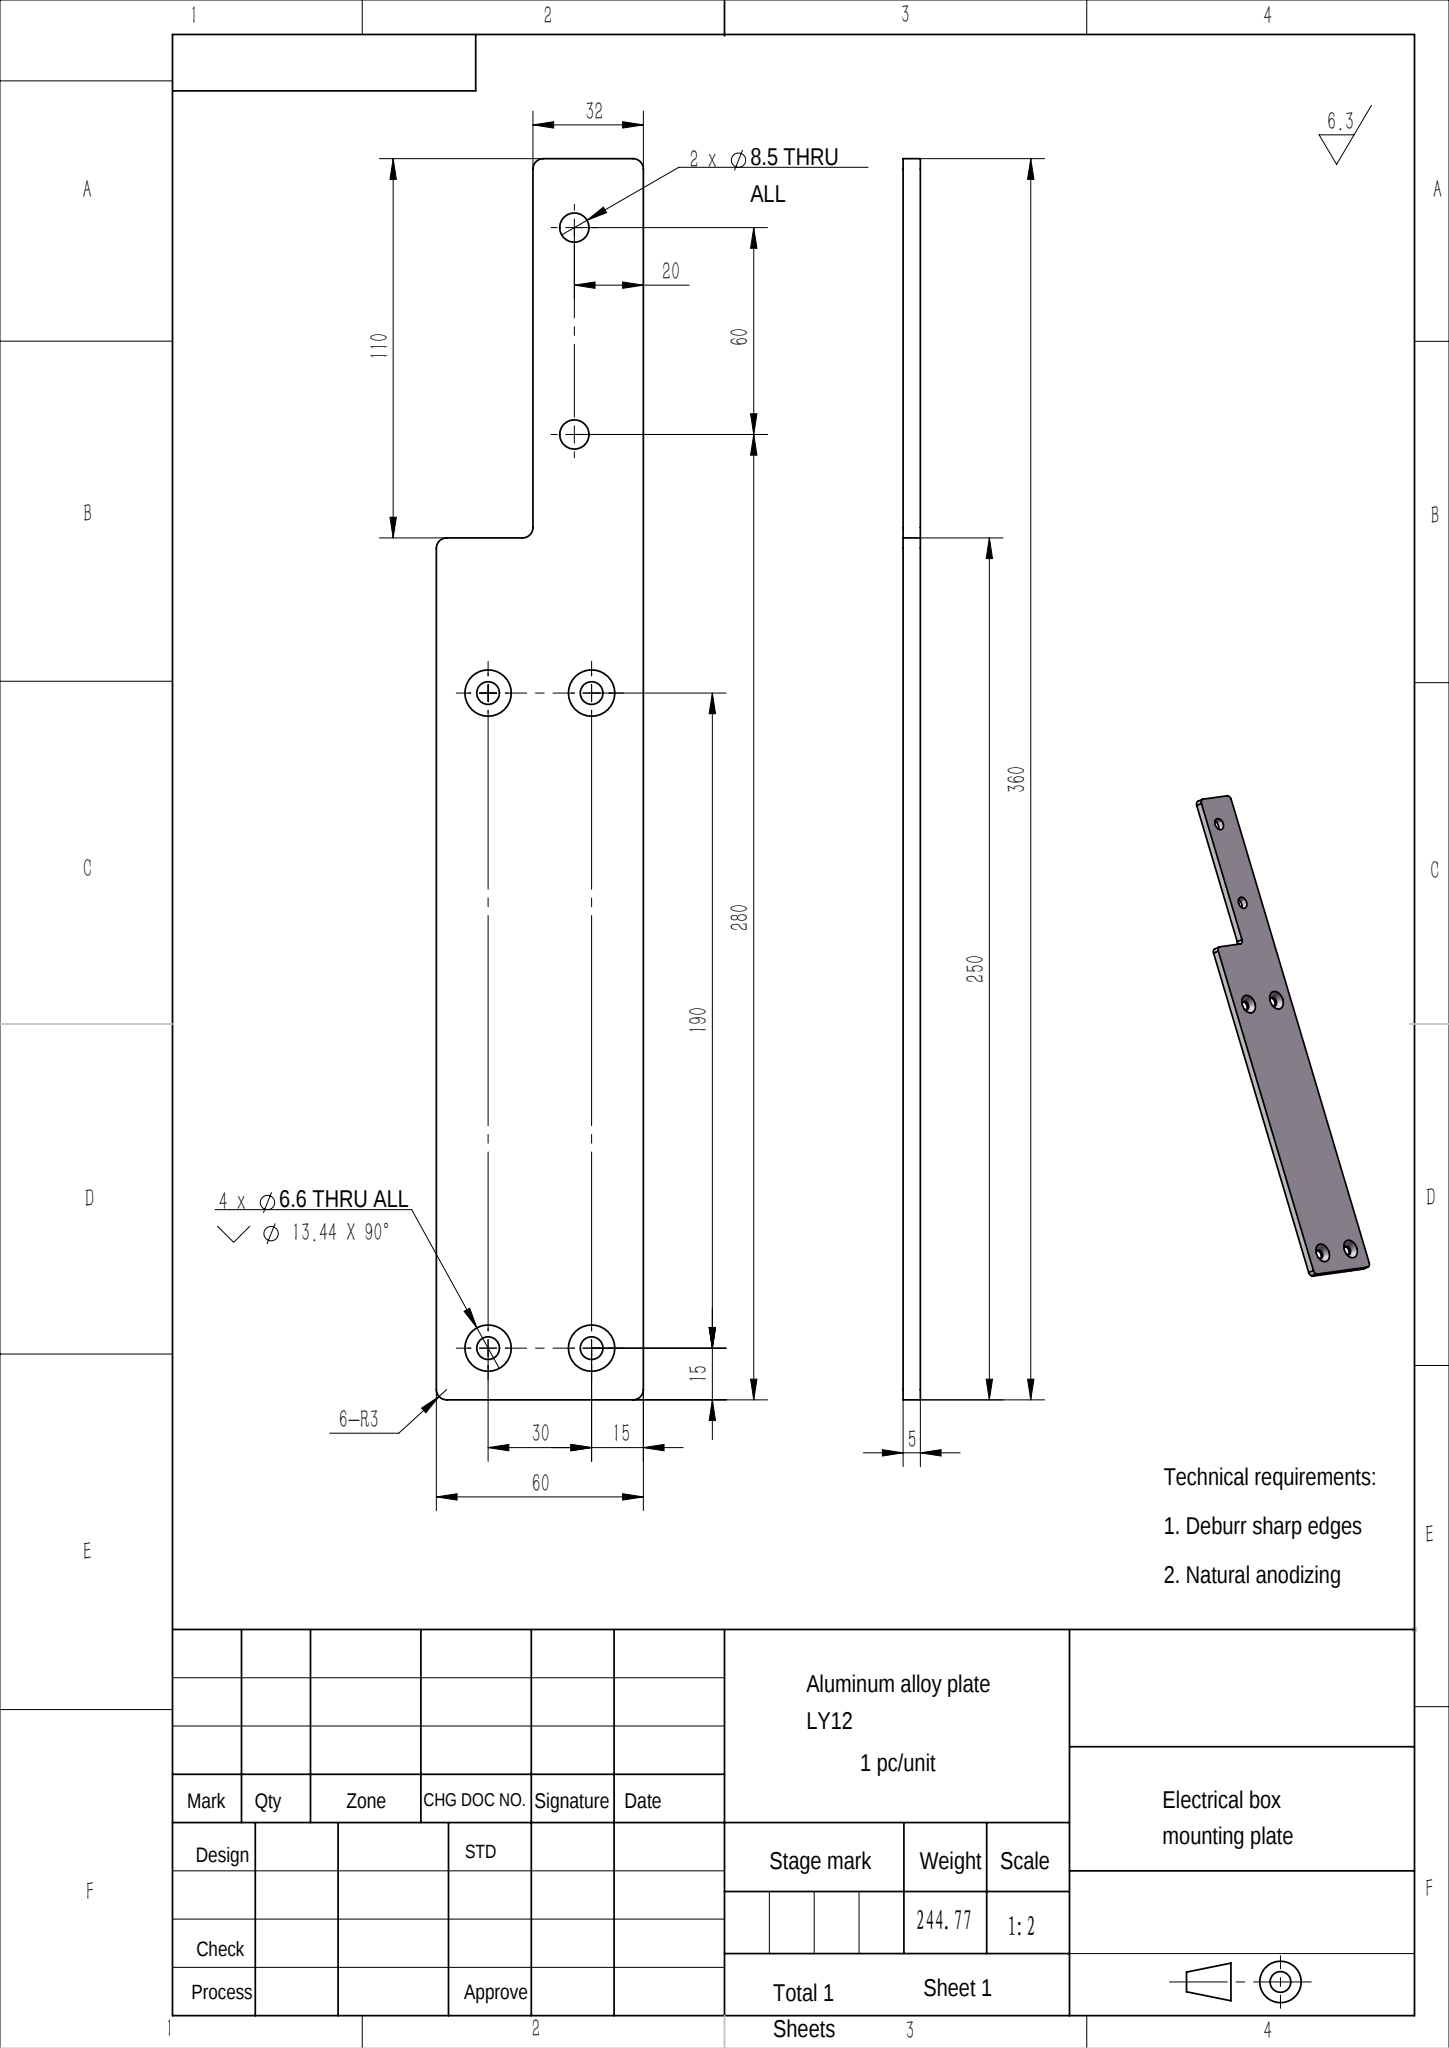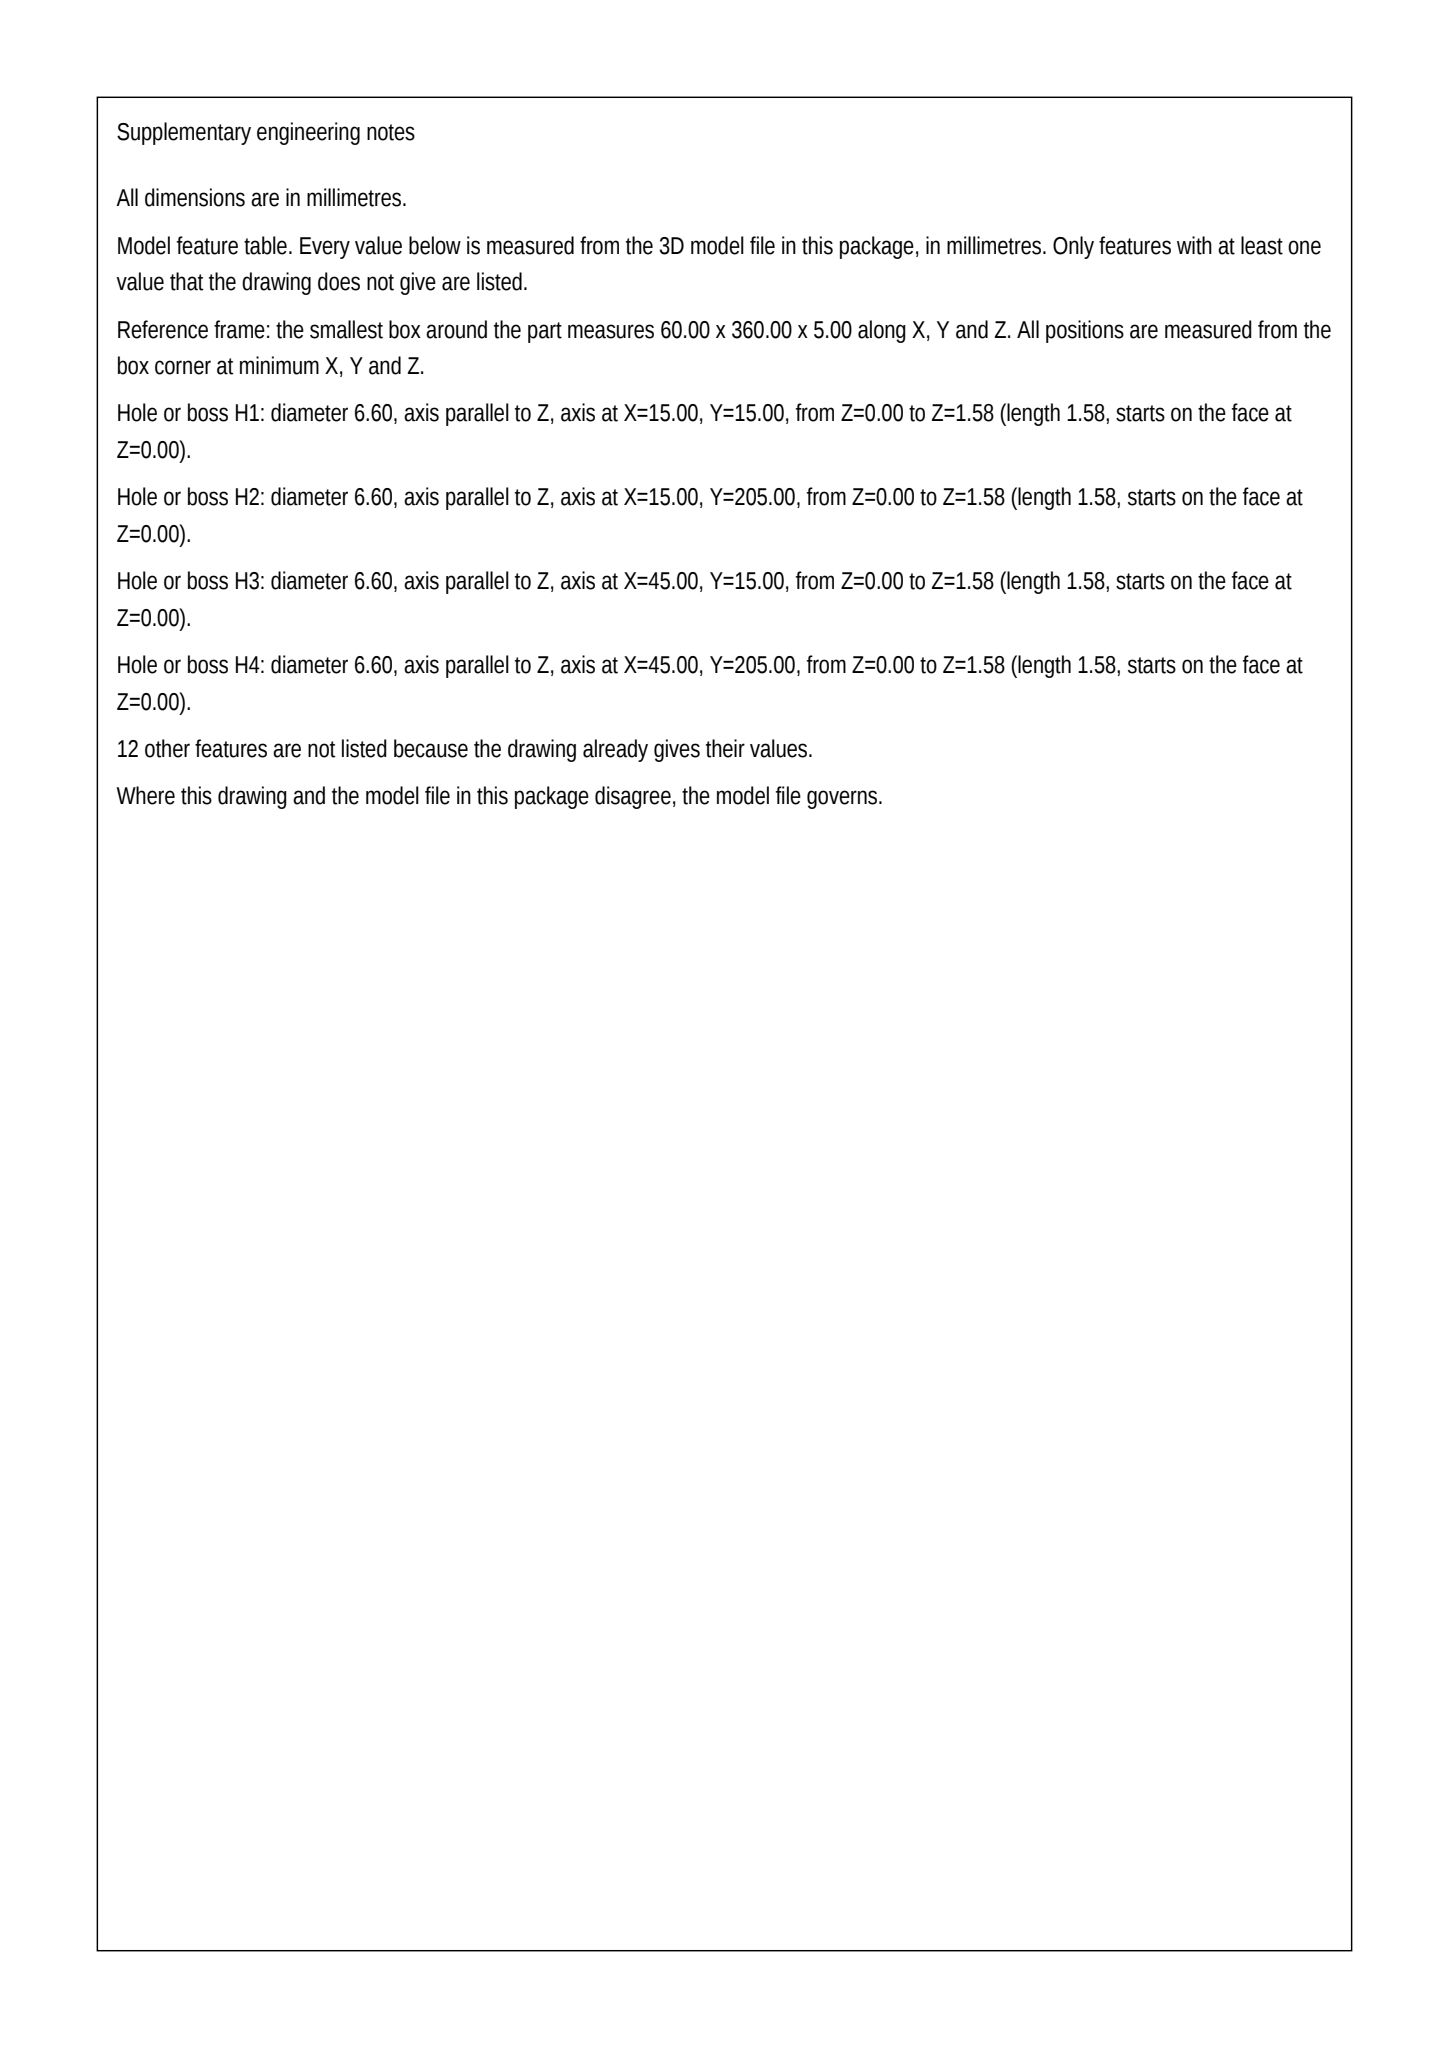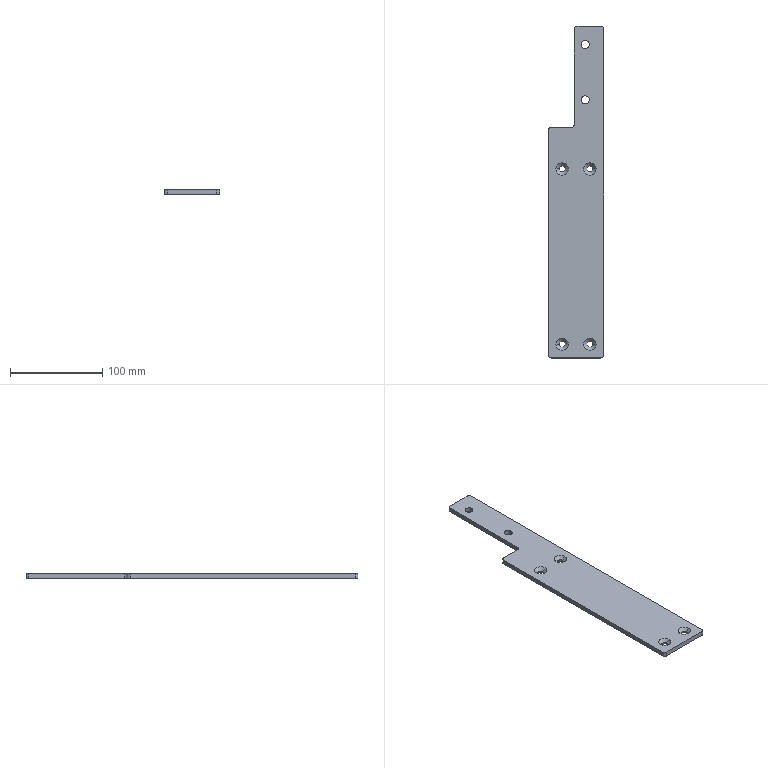Part | SolidWorks | mm | material Aluminum alloy plate LY12 | 1 solid | 34 faces | box 60 x 360 x 5 mm | volume 90657 mm3 | cylinder 18 | cone 8 | plane 8 | commonest cylinder face diameters 6.6 x8 6 x6 8.5 x4